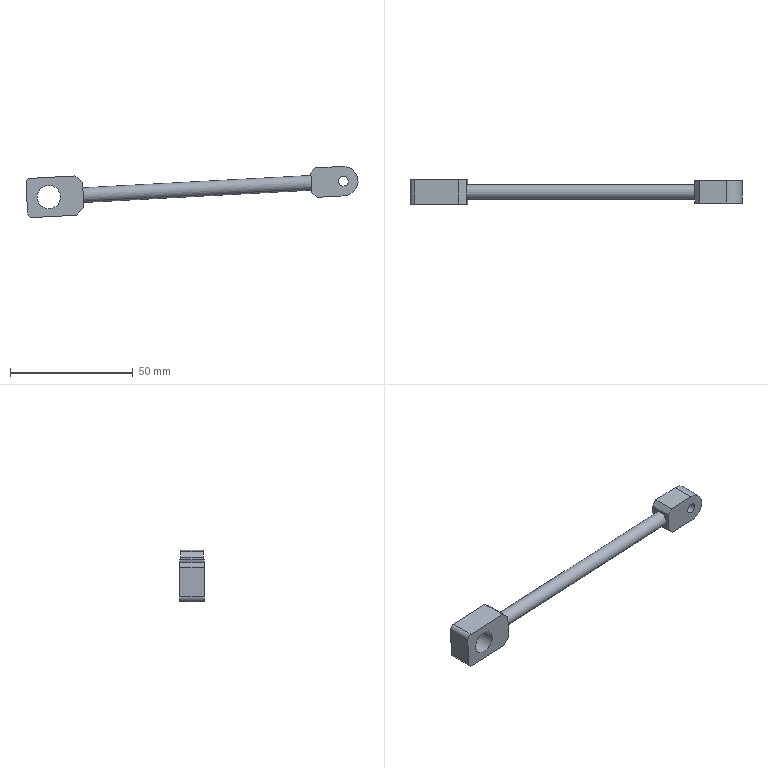Component | NX | CONNECTING_ROD_1 | 1 solid | 21 faces | volume 7257 mm3 | plane 15 | cylinder 6 | commonest cylinder face diameters 4 x3 6 x1 12 x1 9.5 x1